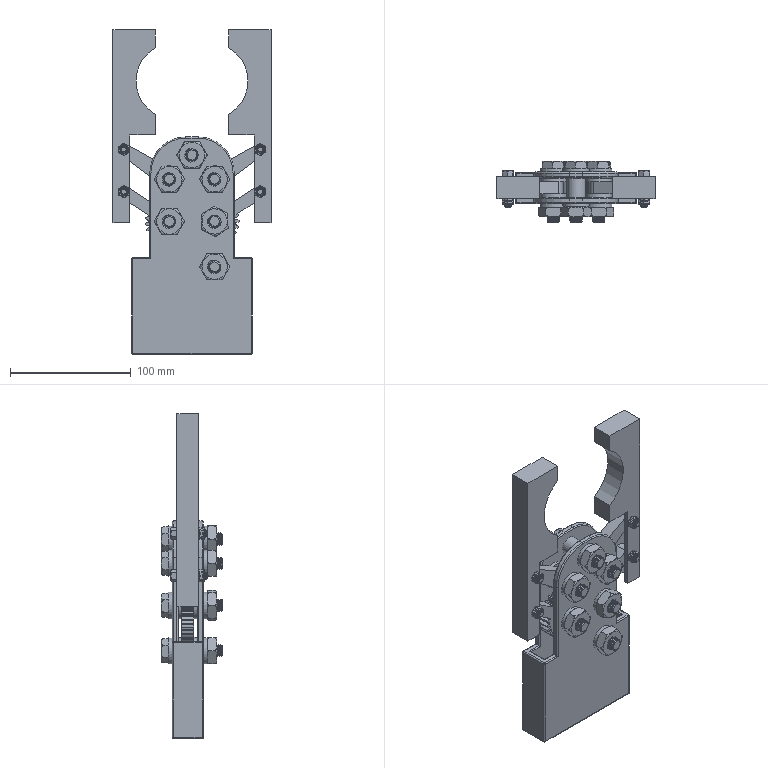Assembly | NX | mm | 54 component files | 64 solids | 1239 faces | box 130.85 x 51 x 268.75 mm | volume 391735 mm3 | spline 520 | cylinder 351 | plane 308 | torus 38 | cone 14 | sphere 8 | commonest cylinder face diameters 10 x115 33.7 x96 6 x51 2 x36 22 x24 12 x6 8.5 x6 60 x4
Bill of materials:
unnamed part 1 | 2 |  | Flat spur-gear-like disc with straight external teeth around its edge and one plain round hole through the center; no hub or web recess.
unnamed part 2 | 2 |  | Flat tapered link or lever plate with rounded ends and one round through hole at each end; the hole at the wide end is bigger than the one at the narrow end.
unnamed part 3 | 2 |  | Flat, uniformly thick plate with a stepped L-like outline: a wider upper section with a semicircular notch cut into one side edge, and a narrower lower leg with two small round through holes.
unnamed part 4 | 4 |  | Hex-head bolt with a long plain shank and a modelled external thread on the end part of the shank.
unnamed part 5 | 1 |  | Plain thick-walled cylindrical tube or sleeve with a smooth round bore running straight through.
unnamed part 6 | 4 |  | Elongated hexagonal nut-like body, longer than it is wide across the flats, with a modelled internal thread in the through bore and chamfered or rounded ends.
unnamed part 7 | 1 |  | Clevis- or fork-style bracket: a rectangular hollow (channel-like) base with two parallel flat plates rising from it, each plate with a rounded top and a pattern of round through holes.
unnamed part 8 | 2 |  | Single flat body combining a spur-gear-like toothed disc with an integral straight arm that ends in a rounded eye with a round hole; the gear disc has its own central round hole.
unnamed part 9 | 6 |  | Hex-head bolt with a plain cylindrical shank and a modelled external thread on the end part.
unnamed part 10 | 24 |  | Flat annular ring (washer-like disc) with a central round hole and constant thickness.
unnamed part 11 | 6 |  | Standard-proportion hexagonal nut with a modelled internal thread in the central bore and chamfered corners on both faces.
Mates:
1. concentric | JJZ-002 2 edge | JJZ-010 24 edge
2. concentric | JJZ-002 1 edge | JJZ-010 21 edge
3. concentric | JJZ-003 2 edge | JJZ-010 22 edge
4. concentric | JJZ-010 23 edge | JJZ-003 1 edge
5. concentric | JJZ-004 2 edge | JJZ-002 1 edge
6. concentric | JJZ-004 2 edge | JJZ-003 2 edge
7. concentric | JJZ-004 1 edge | JJZ-002 2 edge
8. concentric | JJZ-004 1 edge | JJZ-003 1 edge
9. parallel | JJZ-004 1 edge | JJZ-004 2 edge
10. concentric | JJZ-006 6 edge | JJZ-010 16 edge
11. concentric | JJZ-010 15 edge | JJZ-005 6 edge
12. concentric | JJZ-005 5 edge | JJZ-010 13 edge
13. concentric | JJZ-010 12 edge | JJZ-005 4 edge
14. concentric | JJZ-010 14 edge | JJZ-005 3 edge
15. concentric | JJZ-006 5 edge | JJZ-010 9 edge
16. concentric | JJZ-010 11 edge | JJZ-006 4 edge
17. concentric | JJZ-010 10 edge | JJZ-006 3 edge
18. concentric | JJZ-001 1 edge | JJZ-010 16 edge
19. concentric | JJZ-010 8 edge | JJZ-001 1 edge
20. fix | JJZ-001 1 component
21. concentric | JJZ-001 1 edge | JJZ-010 7 edge
22. concentric | JJZ-001 1 edge | JJZ-010 6 edge
23. concentric | JJZ-001 1 edge | JJZ-010 5 edge
24. concentric | JJZ-005 2 edge | JJZ-010 6 edge
25. concentric | JJZ-010 5 edge | JJZ-005 1 edge
26. concentric | JJZ-006 2 edge | JJZ-010 7 edge
27. concentric | JJZ-006 1 edge | JJZ-010 8 edge
28. concentric | JJZ-001 1 edge | JJZ-010 4 edge
29. concentric | JJZ-001 1 edge | JJZ-010 3 edge
30. concentric | JJZ-011 2 edge | JJZ-010 4 edge
31. concentric | JJZ-007 1 edge | JJZ-001 1 edge
32. concentric | JJZ-004 2 edge | JJZ-008 4 edge
33. concentric | JJZ-004 1 edge | JJZ-008 3 edge
34. concentric | JJZ-004 1 edge | JJZ-008 2 edge
35. concentric | JJZ-008 1 edge | JJZ-004 2 edge
36. concentric | JJZ-009 4 edge | JJZ-004 2 edge
37. concentric | JJZ-009 3 edge | JJZ-004 1 edge
38. concentric | JJZ-009 2 edge | JJZ-004 1 edge
39. concentric | JJZ-009 1 edge | JJZ-004 2 edge
40. concentric | JJZ-010 2 edge | JJZ-001 1 edge
41. concentric | JJZ-010 1 edge | JJZ-001 1 edge
42. concentric | JJZ-011 1 edge | JJZ-010 1 edge